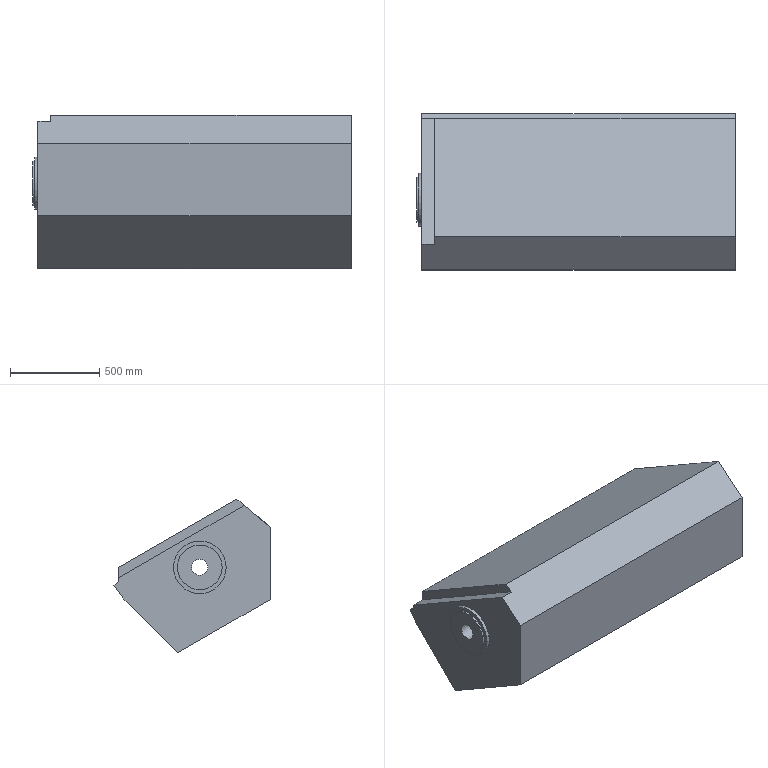Component | NX | SIM15_GEGENSPINDEL | 1 solid | 17 faces | volume 784988475 mm3 | plane 14 | cylinder 3 | commonest cylinder face diameters 295 x1 250 x1 90 x1